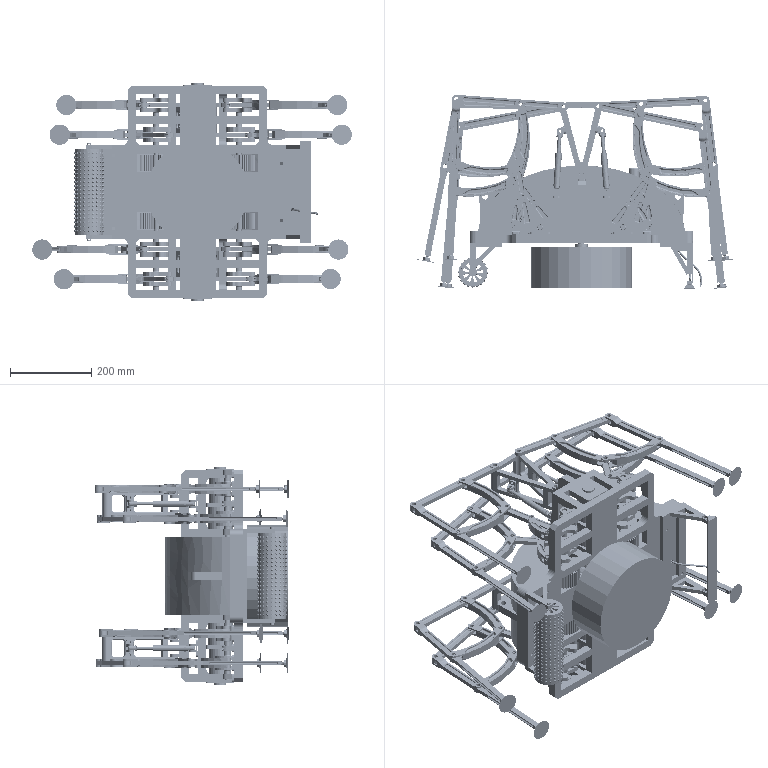Assembly | SolidWorks | mm | 149 component files | 164 solids | 12873 faces | box 787.16 x 478.96 x 537 mm | volume 15869693 mm3 | cylinder 5703 | plane 3151 | torus 1330 | cone 1064 | sphere 1040 | spline 585 | commonest cylinder face diameters 5 x964 10 x524 29.6 x390 32 x336 4 x256 6.25 x256 2 x224 3 x200
Bill of materials:
AxisSeat | 8 |  | Rounded-rectangular flange plate with two through-holes, from which a perpendicular tapered lug projects; the lug ends in a rounded boss with a large through-bore, giving a T-shaped side profile.
BallJointRod | 8 |  | Faceted sphere joined by a short cylindrical neck to a roughly square plate; the plate has a concave curved face toward the sphere and a slotted/stepped edge profile forming two parallel flanges at the back.
BallJointRodUpperPressurePlate | 8 |  | Thin rectangular plate with stepped edge profile: a wider central tongue on one face and offset tabs at the ends, producing a T-slot or tongue-like cross-section.
Rolling bearings 6302 GB 276-94 | 4 |  | Annular rolling-element unit resembling an open radial ball bearing: a plain outer ring and a plain inner ring, concentric, with a ring of spherical balls in the gap between them.
CarBody | 1 |  | Complex frame-like model: a cross-shaped plate with multiple rectangular windows, central plate with a large hole and bolt-hole pattern, stand-off rods, side brackets with triangular gussets and end eyes, a block with a cylindrical protrusion, and flexible cable-like curves.
CleaningCylinder | 1 | Flexible Polyurethane Foam | Short solid cylindrical disc with a small coaxial cylindrical pin protruding from one face.
ConnectingRod1 | 8 |  | Long slightly tapered flat bar/link with a rounded end containing a through-hole, a second through-hole midway, two shallow elongated pockets, and a semicircular cutout at the wider end flanked by small transverse holes.
ConnectingRod1-1 | 8 |  | Half-ring/saddle block: a thick curved body with a semicircular cutout, with angled or oblique holes passing through the outer curved face.
CrankshaftSeat | 8 |  | Pillow-block-like bracket: rounded-rectangular base with two through-holes at the ends and a central tapered upright with a rounded top holding a large through-bore; base underside has a shallow relief.
Cylinder | 1 |  | Cylindrical roller with a regular array of small hemispherical bumps on the outer surface, spoked open end faces (wedge-shaped windows around a hub), and a small shaft extending from both ends with small cross-holes near the shaft tips.
CylinderAxis | 4 |  | Slender cylindrical rod with an enlarged collar near one end, ending in a flat-sided tang/eye with a transverse through-hole.
CylinderBarrel | 4 |  | Cylindrical tube/body with a stepped collar near one end and a flat-sided eye end with a transverse through-hole; the opposite end appears open (hollow).
GearedMotor | 3 |  | Stacked column of two cylindrical bodies separated by square rounded-corner flanges, with a square bottom flange having corner holes, a short round boss on top, and a stepped small shaft at the bottom.
HydraulicCylinderSeat | 8 |  | Bracket: rectangular plate with rounded corners, two through-holes near its ends, and two parallel lugs sticking out from the middle. Each lug has a rounded tip and a through-hole, forming a clevis.
Leg | 8 |  | Long, slender flat bar. One end is forked into a clevis with a cross hole. There is a hole partway along the bar, a long recessed groove on the face, and a notched or grooved far end.
MainCrankshaft | 4 |  | Shaft shaped like a crankshaft: a central round shaft carrying two pairs of lobed webs. Each pair is joined by an offset cylindrical pin, and stepped journals run along the axis.
MiddleCrankshaftSeat | 4 |  | Pillow-block-style mount: base flange with rounded ends and two mounting holes, carrying a raised block with a rounded top. The block has a large through-bore parallel to the base.
RockerArm | 8 |  | Curved link arm with a forked (clevis) end at each end. Each end has paired holes, and there is a long pocket along the curved web.
ScaleInner1 | 8 |  | Curved arm with a forked end at each end and an end hole in each fork. A shaped recessed pocket runs along the curved body, and the body narrows near one end.
ScaleInner2 | 8 |  | Curved link with a forked end at each end and a hole in each tine. A shallow elongated recess runs along the top face.
ScaleInner3 | 8 |  | Straight, flat bar with rounded ends. It has a hole at each end, a central hole, and two long shallow recesses on one face.
Scraper | 1 |  | Long, slender prismatic bar whose cross-section is stepped: a narrow rectangle on top of a trapezoidal base. The top-left view shows a second offset trapezoidal outline. Small rectangular notches sit near each end.
Spring | 2 |  | Helical coil of round wire with roughly constant diameter and pitch, open coil spacing, and plain cut ends.
GB - Spur gear 2M 37T 20PA 37FW ---S37A75H50L16.0S1 | 1 |  | Spur gear: a flat cylindrical disc with straight external teeth all around and a central circular bore with a single rectangular keyway.
spur gear_gb | 4 |  | Spur gear: a flat cylindrical disc with straight external teeth and a fairly small central circular bore with a single rectangular keyway.
GB - Spur gear 2M 40T 20PA 40FW ---S40A75H50L12.0S1 | 4 |  | Spur gear: a flat cylindrical disc with straight external teeth (apparently slightly more and finer than in the other gears) and a small central circular bore with a single rectangular keyway.
SuctionCup | 8 |  | Thin circular disc with a small polygonal or rectangular boss on one face. The edge appears thin and possibly tapered.
TopCover | 1 |  | Thin-walled shroud or housing: a curved (arched) shell enclosed by end walls, with a rectangular perimeter flange around its open face. The flange has corner tabs with small holes. The lower edge has notches and a central U-shaped slot, and there is one hole in the curved wall.
UpperAxisSeat | 4 |  | Clevis-style double-lug bracket: a flat rectangular base plate with rounded corners and one through hole near each end, with two parallel, equal lugs standing up from the middle of the plate. Each lug has a rounded end, sides that taper slightly, and a large round hole; the two lug holes appear to share one axis.
VibrationDampingBracket | 2 |  | Lightweighted, truss-like triangular bracket: an open triangular frame, roughly an isosceles outline, with a round hole at each of its three rounded corners. It sits on top of a deeper structure of upright walls with large rectangular openings, diagonal braces and posts. A rectangular web in the middle carries two small holes.
Mates:
1. concentric | ScaleInner1-1 face at (-140.193, -93.224, 219.713) dir (0, 0, -1) r 5 | Leg-1 face at (-140.193, -93.224, 211.463) dir (0, 0, -1) r 5
2. coincident | ScaleInner1-1 face at (-137.996, -126.993, 201.463) dir (0, 0, 1) | Leg-1 face at (-148.968, -330.662, 201.463) dir (0, 0, -1)
3. concentric | ScaleInner1-1 face at (17.789, -104.729, 219.713) dir (0, 0, -1) r 5 | ScaleInner2-1 face at (17.789, -104.729, 215.713) dir (0, 0, -1) r 5
4. coincident | ScaleInner1-1 face at (17.789, -104.729, 197.213) dir (0, 0, 1) | ScaleInner2-1 face at (-85.717, 17.977, 197.213) dir (0, 0, -1)
5. concentric | ScaleInner3-1 face at (-134.342, 65.068, 211.463) dir (0, 0, -1) r 5 | Leg-1 face at (-134.343, 65.068, 211.463) dir (0, 0, -1) r 5
6. coincident | ScaleInner3-1 face at (128.961, 45.893, 211.463) dir (0, 0, 1) | Leg-1 face at (-134.343, 65.068, 211.463) dir (0, 0, -1)
7. concentric | ScaleInner2-1 face at (23.639, 53.563, 215.713) dir (0, 0, -1) r 5 | ScaleInner3-1 face at (23.64, 53.563, 211.463) dir (0, 0, -1) r 5
8. concentric | ConnectingRod1-1 face at (17.789, -104.729, 201.463) dir (0, 0, 1) r 5 | ScaleInner1-1 face at (17.789, -104.729, 219.713) dir (0, 0, -1) r 5
9. coincident | ConnectingRod1-1 face at (39.348, -177.229, 211.463) dir (0, 0, 1) | ScaleInner2-1 face at (51.343, -100.957, 211.463) dir (0, 0, -1)
10. concentric | ConnectingRod1-1 face at (31.955, -256.986, 206.463) dir (-0.1656, 0.9862, 0) r 1.5 | ConnectingRod1-1-1 face at (32.038, -257.479, 206.463) dir (-0.1656, 0.9862, 0) r 1.5
11. concentric | ConnectingRod1-1 face at (54.144, -253.259, 206.463) dir (-0.1656, 0.9862, 0) r 1.5 | ConnectingRod1-1-1 face at (54.227, -253.752, 206.463) dir (-0.1656, 0.9862, 0) r 1.5
12. coincident | ConnectingRod1-1 face at (72.659, -247.614, 213.963) dir (0.1656, -0.9862, 0) | ConnectingRod1-1-1 face at (28.829, -254.976, 201.463) dir (-0.1656, 0.9862, 0)
13. concentric | ConnectingRod1-1 face at (30.212, -178.693, 201.463) dir (0, 0, 1) r 5.625 | RockerArm-1 face at (30.212, -178.693, 217.463) dir (0, 0, -1) r 5.625
14. coincident | ConnectingRod1-1 face at (39.348, -177.229, 211.463) dir (0, 0, 1) | RockerArm-1 face at (67.023, -246.948, 211.463) dir (0, 0, -1)
15. concentric | CarBody-1 face at (174.617, -142.6, 213.713) dir (0, 1, 0) r 3.125 | UpperAxisSeat-1 face at (174.617, -111.1, 213.713) dir (0, -1, 0) r 3.125
16. concentric | CarBody-1 face at (174.617, -142.6, 179.213) dir (0, 1, 0) r 3.125 | UpperAxisSeat-1 face at (174.617, -111.1, 179.213) dir (0, -1, 0) r 3.125
17. coincident | CarBody-1 face at (174.617, -137.6, -8.037) dir (0, 1, 0) | UpperAxisSeat-1 face at (174.617, -137.6, 196.463) dir (0, -1, 0)
18. concentric | VibrationDampingBracket-1 face at (174.617, -120.35, 138.463) dir (0, 0, 1) r 5 | UpperAxisSeat-1 face at (174.617, -120.35, 208.463) dir (0, 0, -1) r 5
19. coincident | VibrationDampingBracket-1 face at (128.96, 45.893, 201.463) dir (0, 0, 1) | UpperAxisSeat-1 face at (174.617, -120.35, 201.463) dir (0, 0, -1)
20. concentric | CarBody-1 face at (174.617, -142.6, 126.213) dir (0, 1, 0) r 3.125 | UpperAxisSeat-2 face at (174.617, -111.1, 126.213) dir (0, -1, 0) r 3.125
21. concentric | CarBody-1 face at (174.617, -142.6, 160.713) dir (0, 1, 0) r 3.125 | UpperAxisSeat-2 face at (174.617, -111.1, 160.713) dir (0, -1, 0) r 3.125
22. coincident | CarBody-1 face at (174.617, -137.6, -8.037) dir (0, 1, 0) | UpperAxisSeat-2 face at (174.617, -137.6, 143.463) dir (0, -1, 0)
23. concentric | CarBody-1 face at (12.617, -274.1, 220.838) dir (0, 1, 0) r 3.125 | AxisSeat-1 face at (12.617, -266.35, 220.838) dir (0, 1, 0) r 4.5
24. concentric | CarBody-1 face at (12.617, -274.1, 192.088) dir (0, 1, 0) r 3.125 | AxisSeat-1 face at (12.617, -266.35, 192.088) dir (0, 1, 0) r 4.5
25. coincident | CarBody-1 face at (449.617, -269.1, -108.037) dir (0, 1, 0) | AxisSeat-1 face at (12.617, -269.1, 206.463) dir (0, -1, 0)
26. concentric | RockerArm-1 face at (12.617, -251.6, 217.463) dir (0, 0, -1) r 5.625 | AxisSeat-1 face at (12.617, -251.6, 201.463) dir (0, 0, 1) r 5.625
27. coincident | RockerArm-1 face at (56.993, -257.493, 211.463) dir (0, 0, -1) | AxisSeat-1 face at (12.617, -251.6, 211.463) dir (0, 0, 1)
28. concentric | ScaleInner3-1 face at (128.961, 45.893, 211.463) dir (0, 0, -1) r 5 | VibrationDampingBracket-1 face at (128.96, 45.893, 138.463) dir (0, 0, 1) r 5
29. concentric | CarBody-1 face at (52.617, -274.1, 242.963) dir (0, 1, 0) r 3.125 | CrankshaftSeat-1 face at (52.617, -269.1, 242.963) dir (0, 1, 0) r 3.125
30. concentric | CarBody-1 face at (92.617, -274.1, 242.963) dir (0, 1, 0) r 3.125 | CrankshaftSeat-1 face at (92.617, -269.1, 242.963) dir (0, 1, 0) r 3.125
31. coincident | CarBody-1 face at (449.617, -269.1, -108.037) dir (0, 1, 0) | CrankshaftSeat-1 face at (72.617, -269.1, 242.963) dir (0, -1, 0)
32. concentric | CarBody-1 face at (52.617, -274.1, 96.963) dir (0, 1, 0) r 3.125 | CrankshaftSeat-2 face at (52.617, -269.1, 96.963) dir (0, 1, 0) r 3.125
33. concentric | CarBody-1 face at (92.617, -274.1, 96.963) dir (0, 1, 0) r 3.125 | CrankshaftSeat-2 face at (92.617, -269.1, 96.963) dir (0, 1, 0) r 3.125
34. coincident | CarBody-1 face at (449.617, -269.1, -108.037) dir (0, 1, 0) | CrankshaftSeat-2 face at (72.617, -269.1, 96.963) dir (0, -1, 0)
35. concentric | MainCrankshaft-1 face at (72.617, -251.6, 247.963) dir (0, 0, -1) r 6.75 | CrankshaftSeat-1 face at (72.617, -251.6, 239.963) dir (0, 0, 1) r 6.75
36. concentric | ConnectingRod1-1 face at (42.635, -252.657, 201.463) dir (0, 0, 1) r 7.5 | MainCrankshaft-1 face at (42.635, -252.657, 213.963) dir (0, 0, -1) r 6.25
37. concentric | Leg-2 face at (-144.409, -161.167, 138.463) dir (0, 0, -1) r 5 | ScaleInner1-2 face at (-144.409, -161.167, 146.713) dir (0, 0, -1) r 5
38. concentric | ScaleInner3-2 face at (-130.399, -3.388, 138.463) dir (0, 0, -1) r 5 | Leg-2 face at (-130.399, -3.388, 138.463) dir (0, 0, -1) r 5
39. coincident | ScaleInner3-2 face at (128.961, 45.893, 138.463) dir (0, 0, 1) | Leg-2 face at (-130.399, -3.388, 138.463) dir (0, 0, -1)
40. concentric | ScaleInner3-2 face at (25.217, 26.181, 138.463) dir (0, 0, -1) r 5 | ScaleInner2-2 face at (25.216, 26.181, 142.713) dir (0, 0, -1) r 5
41. coincident | ScaleInner3-2 face at (128.961, 45.893, 138.463) dir (0, 0, 1) | ScaleInner2-2 face at (25.216, 26.181, 138.463) dir (0, 0, -1)
42. coincident | Leg-2 face at (-165.423, -397.836, 128.463) dir (0, 0, -1) | ScaleInner1-2 face at (-133.59, -193.232, 128.463) dir (0, 0, 1)
43. concentric | ScaleInner1-2 face at (11.207, -131.599, 146.713) dir (0, 0, -1) r 5 | ScaleInner2-2 face at (11.207, -131.599, 142.713) dir (0, 0, -1) r 5
44. concentric | ConnectingRod1-2 face at (95.201, -259.379, 133.463) dir (-0.6093, 0.793, 0) r 1.5 | ConnectingRod1-1-2 face at (95.505, -259.776, 133.463) dir (-0.6093, 0.793, 0) r 1.5
45. concentric | ConnectingRod1-2 face at (113.042, -245.671, 133.463) dir (-0.6093, 0.793, 0) r 1.5 | ConnectingRod1-1-2 face at (113.347, -246.067, 133.463) dir (-0.6093, 0.793, 0) r 1.5
46. coincident | ConnectingRod1-2 face at (126.739, -231.994, 140.963) dir (0.6093, -0.793, 0) | ConnectingRod1-1-2 face at (91.497, -259.072, 128.463) dir (-0.6093, 0.793, 0)
47. concentric | ConnectingRod1-2 face at (56.903, -191.071, 128.463) dir (0, 0, 1) r 5.625 | RockerArm-2 face at (56.903, -191.071, 144.463) dir (0, 0, -1) r 5.625
48. coincident | ConnectingRod1-2 face at (64.282, -185.489, 138.463) dir (0, 0, 1) | RockerArm-2 face at (64.626, -268.234, 138.463) dir (0, 0, -1)
49. concentric | ConnectingRod1-2 face at (11.207, -131.599, 128.463) dir (0, 0, 1) r 5 | ScaleInner2-2 face at (11.207, -131.599, 142.713) dir (0, 0, -1) r 5
50. coincident | ConnectingRod1-2 face at (64.282, -185.489, 138.463) dir (0, 0, 1) | ScaleInner2-2 face at (44.911, -129.563, 138.463) dir (0, 0, -1)
51. concentric | VibrationDampingBracket-1 face at (128.96, 45.893, 138.463) dir (0, 0, 1) r 5 | ScaleInner3-2 face at (128.961, 45.893, 138.463) dir (0, 0, -1) r 5
52. coincident | VibrationDampingBracket-1 face at (128.96, 45.893, 138.463) dir (0, 0, -1) | ScaleInner3-2 face at (128.961, 45.893, 138.463) dir (0, 0, 1)
53. concentric | MainCrankshaft-1 face at (102.598, -250.543, 140.963) dir (0, 0, -1) r 6.25 | ConnectingRod1-2 face at (102.598, -250.543, 128.463) dir (0, 0, 1) r 7.5
54. concentric | CarBody-1 face at (12.617, -274.1, 147.838) dir (0, 1, 0) r 3.125 | AxisSeat-2 face at (12.617, -266.35, 147.838) dir (0, 1, 0) r 4.5
55. concentric | CarBody-1 face at (12.617, -274.1, 119.088) dir (0, 1, 0) r 3.125 | AxisSeat-2 face at (12.617, -242.85, 119.088) dir (0, -1, 0) r 3.125
56. coincident | CarBody-1 face at (449.617, -269.1, -108.037) dir (0, 1, 0) | AxisSeat-2 face at (12.617, -269.1, 133.463) dir (0, -1, 0)
57. concentric | RockerArm-2 face at (12.617, -251.6, 144.463) dir (0, 0, -1) r 5.625 | AxisSeat-2 face at (12.617, -251.6, 138.463) dir (0, 0, -1) r 5.625
58. concentric | CarBody-1 face at (48.617, -274.1, 169.963) dir (0, 1, 0) r 3.125 | MiddleCrankshaftSeat-1 face at (48.617, -262.85, 169.963) dir (0, -1, 0) r 3.125
59. concentric | CarBody-1 face at (96.617, -274.1, 169.963) dir (0, 1, 0) r 3.125 | MiddleCrankshaftSeat-1 face at (96.617, -262.85, 169.963) dir (0, -1, 0) r 3.125
60. coincident | CarBody-1 face at (449.617, -269.1, -108.037) dir (0, 1, 0) | MiddleCrankshaftSeat-1 face at (72.617, -269.1, 169.963) dir (0, -1, 0)
61. coincident | MainCrankshaft-1 face at (72.617, -251.6, 106.963) dir (0, 0, -1) | CrankshaftSeat-2 face at (47.617, -262.85, 106.963) dir (0, 0, 1)
62. concentric | ConnectingRod1-3 face at (54.284, -247.009, -149.537) dir (-0.3125, 0.9499, 0) r 1.5 | ConnectingRod1-1-5 face at (54.44, -247.484, -149.537) dir (-0.3125, 0.9499, 0) r 1.5
63. concentric | ConnectingRod1-3 face at (32.91, -254.04, -149.537) dir (-0.3125, 0.9499, 0) r 1.5 | ConnectingRod1-1-5 face at (33.067, -254.515, -149.537) dir (-0.3125, 0.9499, 0) r 1.5
64. coincident | ConnectingRod1-3 face at (71.736, -238.637, -142.037) dir (0.3125, -0.9499, 0) | ConnectingRod1-1-5 face at (49.94, -245.806, -154.537) dir (-0.3125, 0.9499, 0)
65. concentric | ConnectingRod1-1-4 face at (235.786, -248.339, 206.463) dir (0.5913, 0.8065, 0) r 1.5 | ConnectingRod1-4 face at (236.082, -247.936, 206.463) dir (0.5913, 0.8065, 0) r 1.5
66. concentric | ConnectingRod1-1-4 face at (253.932, -261.642, 206.463) dir (0.5913, 0.8065, 0) r 1.5 | ConnectingRod1-4 face at (254.227, -261.239, 206.463) dir (0.5913, 0.8065, 0) r 1.5
67. coincident | ConnectingRod1-1-4 face at (240.584, -248.137, 211.463) dir (0.5913, 0.8065, 0) | ConnectingRod1-4 face at (222.08, -234.571, 198.963) dir (-0.5913, -0.8065, 0)
68. concentric | Leg-3 face at (-162.383, -100.897, -144.537) dir (0, 0, -1) r 5 | ScaleInner1-3 face at (-162.383, -100.897, -136.287) dir (0, 0, -1) r 5
69. coincident | Leg-3 face at (-207.807, -334.115, -144.537) dir (0, 0, 1) | ScaleInner1-3 face at (-158.75, -134.542, -144.537) dir (0, 0, -1)
70. concentric | ScaleInner2-3 face at (-4.055, -105.661, -140.287) dir (0, 0, -1) r 5 | ScaleInner1-3 face at (-4.055, -105.661, -136.287) dir (0, 0, -1) r 5
71. coincident | ScaleInner2-3 face at (-87.318, 31.589, -140.287) dir (0, 0, 1) | ScaleInner1-3 face at (-4.055, -105.661, -140.287) dir (0, 0, -1)
72. concentric | ScaleInner3-3 face at (-132.1, 54.581, -144.537) dir (0, 0, -1) r 5 | Leg-3 face at (-132.1, 54.581, -144.537) dir (0, 0, -1) r 5
73. coincident | ScaleInner3-3 face at (131.781, 46.642, -144.537) dir (0, 0, 1) | Leg-3 face at (-132.1, 54.581, -144.537) dir (0, 0, -1)
74. concentric | ScaleInner3-3 face at (26.228, 49.818, -144.537) dir (0, 0, -1) r 5 | ScaleInner2-3 face at (26.228, 49.818, -140.287) dir (0, 0, -1) r 5
75. concentric | ScaleInner2-3 face at (-4.055, -105.661, -140.287) dir (0, 0, -1) r 5 | ConnectingRod1-3 face at (-4.055, -105.661, -154.537) dir (0, 0, 1) r 5
76. coincident | ScaleInner2-3 face at (29.679, -107.129, -144.537) dir (0, 0, -1) | ConnectingRod1-3 face at (28.191, -174.08, -144.537) dir (0, 0, 1)
77. concentric | CarBody-1 face at (174.617, -142.6, -142.287) dir (0, 1, 0) r 3.125 | UpperAxisSeat-3 face at (174.617, -111.1, -142.287) dir (0, -1, 0) r 3.125
78. concentric | CarBody-1 face at (174.617, -142.6, -176.787) dir (0, 1, 0) r 3.125 | UpperAxisSeat-3 face at (174.617, -111.1, -176.787) dir (0, -1, 0) r 3.125
79. coincident | CarBody-1 face at (174.617, -137.6, -8.037) dir (0, 1, 0) | UpperAxisSeat-3 face at (174.617, -137.6, -159.537) dir (0, -1, 0)
80. concentric | CarBody-1 face at (174.617, -142.6, -195.287) dir (0, 1, 0) r 3.125 | UpperAxisSeat-4 face at (174.617, -111.1, -195.287) dir (0, -1, 0) r 3.125
81. concentric | CarBody-1 face at (174.617, -142.6, -229.787) dir (0, 1, 0) r 3.125 | UpperAxisSeat-4 face at (174.617, -111.1, -229.787) dir (0, -1, 0) r 3.125
82. coincident | CarBody-1 face at (174.617, -137.6, -8.037) dir (0, 1, 0) | UpperAxisSeat-4 face at (174.617, -137.6, -212.537) dir (0, -1, 0)
83. concentric | UpperAxisSeat-4 face at (174.617, -120.35, -224.537) dir (0, 0, 1) r 5 | VibrationDampingBracket-2 face at (174.617, -120.35, -217.537) dir (0, 0, 1) r 5
84. coincident | UpperAxisSeat-4 face at (174.617, -120.35, -217.537) dir (0, 0, 1) | VibrationDampingBracket-2 face at (131.78, 46.642, -217.537) dir (0, 0, -1)
85. concentric | ScaleInner3-3 face at (131.781, 46.642, -144.537) dir (0, 0, -1) r 5 | VibrationDampingBracket-2 face at (131.78, 46.642, -217.537) dir (0, 0, 1) r 5
86. coincident | ScaleInner3-3 face at (131.781, 46.642, -154.537) dir (0, 0, -1) | VibrationDampingBracket-2 face at (131.78, 46.642, -154.537) dir (0, 0, 1)
87. coincident | Leg-4 face at (-127.342, -3.874, -217.537) dir (0, 0, -1) | ScaleInner3-4 face at (131.781, 46.642, -217.537) dir (0, 0, 1)
88. concentric | Leg-4 face at (-127.342, -3.874, -217.537) dir (0, 0, -1) r 5 | ScaleInner3-4 face at (-127.341, -3.874, -217.537) dir (0, 0, -1) r 5
89. concentric | VibrationDampingBracket-2 face at (131.78, 46.642, -217.537) dir (0, 0, 1) r 5 | ScaleInner3-4 face at (131.781, 46.642, -217.537) dir (0, 0, -1) r 5
90. coincident | VibrationDampingBracket-2 face at (131.78, 46.642, -217.537) dir (0, 0, -1) | ScaleInner3-4 face at (131.781, 46.642, -217.537) dir (0, 0, 1)
91. concentric | ConnectingRod1-3 face at (19.381, -176.905, -154.537) dir (0, 0, 1) r 5.625 | RockerArm-4 face at (19.381, -176.905, -138.037) dir (0, 0, -1) r 5.625
92. coincident | ConnectingRod1-3 face at (28.191, -174.08, -154.537) dir (0, 0, -1) | RockerArm-4 face at (65.761, -239.055, -154.537) dir (0, 0, 1)
93. concentric | CarBody-1 face at (52.617, -274.1, -113.037) dir (0, 1, 0) r 3.125 | CrankshaftSeat-3 face at (52.617, -269.1, -113.037) dir (0, 1, 0) r 3.125
94. concentric | CarBody-1 face at (92.617, -274.1, -113.037) dir (0, 1, 0) r 3.125 | CrankshaftSeat-3 face at (92.617, -269.1, -113.037) dir (0, 1, 0) r 3.125
95. coincident | CarBody-1 face at (449.617, -269.1, -108.037) dir (0, 1, 0) | CrankshaftSeat-3 face at (72.617, -269.1, -113.037) dir (0, -1, 0)
96. concentric | CarBody-1 face at (52.617, -274.1, -259.037) dir (0, 1, 0) r 3.125 | CrankshaftSeat-4 face at (52.617, -269.1, -259.037) dir (0, 1, 0) r 3.125
97. concentric | CarBody-1 face at (92.617, -274.1, -259.037) dir (0, 1, 0) r 3.125 | CrankshaftSeat-4 face at (92.617, -269.1, -259.037) dir (0, 1, 0) r 3.125
98. coincident | CarBody-1 face at (449.617, -269.1, -108.037) dir (0, 1, 0) | CrankshaftSeat-4 face at (72.617, -269.1, -259.037) dir (0, -1, 0)
99. concentric | CarBody-1 face at (12.617, -274.1, -135.162) dir (0, 1, 0) r 3.125 | AxisSeat-3 face at (12.617, -266.35, -135.162) dir (0, 1, 0) r 4.5
100. concentric | CarBody-1 face at (12.617, -274.1, -163.912) dir (0, 1, 0) r 3.125 | AxisSeat-3 face at (12.617, -242.85, -163.912) dir (0, -1, 0) r 3.125
101. coincident | CarBody-1 face at (449.617, -269.1, -108.037) dir (0, 1, 0) | AxisSeat-3 face at (12.617, -269.1, -149.537) dir (0, -1, 0)
102. concentric | CarBody-1 face at (12.617, -274.1, -236.912) dir (0, 1, 0) r 3.125 | AxisSeat-4 face at (12.617, -242.85, -236.912) dir (0, -1, 0) r 3.125
103. concentric | CarBody-1 face at (12.617, -274.1, -208.162) dir (0, 1, 0) r 3.125 | AxisSeat-4 face at (12.617, -242.85, -208.162) dir (0, -1, 0) r 3.125
104. coincident | CarBody-1 face at (449.617, -269.1, -108.037) dir (0, 1, 0) | AxisSeat-4 face at (12.617, -269.1, -222.537) dir (0, -1, 0)
105. concentric | RockerArm-4 face at (12.617, -251.6, -138.037) dir (0, 0, -1) r 5.625 | AxisSeat-3 face at (12.617, -251.6, -144.537) dir (0, 0, -1) r 5.625
106. concentric | CrankshaftSeat-4 face at (72.617, -251.6, -262.037) dir (0, 0, 1) r 6.75 | MainCrankshaft-3 face at (72.617, -251.6, -264.037) dir (0, 0, 1) r 6.75
107. concentric | ConnectingRod1-1-5 face at (42.816, -248.15, -154.537) dir (0, 0, 1) r 7.5 | MainCrankshaft-3 face at (42.816, -248.15, -157.037) dir (0, 0, 1) r 6.25
108. concentric | CarBody-1 face at (48.617, -274.1, -186.037) dir (0, 1, 0) r 3.125 | MiddleCrankshaftSeat-2 face at (48.617, -262.85, -186.037) dir (0, -1, 0) r 3.125
109. concentric | CarBody-1 face at (96.617, -274.1, -186.037) dir (0, 1, 0) r 3.125 | MiddleCrankshaftSeat-2 face at (96.617, -262.85, -186.037) dir (0, -1, 0) r 3.125
110. coincident | CarBody-1 face at (449.617, -269.1, -108.037) dir (0, 1, 0) | MiddleCrankshaftSeat-2 face at (72.617, -269.1, -186.037) dir (0, -1, 0)
111. width | MainCrankshaft-3 face at (72.617, -251.6, -178.537) dir (0, 0, -1) | MainCrankshaft-3 face at (72.617, -251.6, -193.537) dir (0, 0, 1) | MiddleCrankshaftSeat-2 face at (72.617, -251.6, -192.287) dir (0, 0, -1) | MiddleCrankshaftSeat-2 face at (72.617, -251.6, -179.787) dir (0, 0, 1)
112. concentric | ScaleInner1-5 face at (490.257, -164.548, 193.213) dir (0, 0, 1) r 5 | Leg-5 face at (490.257, -164.548, 201.463) dir (0, 0, 1) r 5
113. coincident | ScaleInner1-5 face at (478.742, -196.369, 201.463) dir (0, 0, 1) | Leg-5 face at (518.366, -400.479, 201.463) dir (0, 0, -1)
114. concentric | ScaleInner2-5 face at (335.321, -131.599, 215.713) dir (0, 0, -1) r 5 | ScaleInner1-5 face at (335.321, -131.599, 193.213) dir (0, 0, 1) r 5
115. coincident | ScaleInner2-5 face at (437.845, -79.504, 197.213) dir (0, 0, -1) | ScaleInner1-5 face at (335.321, -131.599, 197.213) dir (0, 0, 1)
116. concentric | ScaleInner3-5 face at (471.517, -7.26, 201.463) dir (0, 0, 1) r 5 | Leg-5 face at (471.517, -7.26, 201.463) dir (0, 0, 1) r 5
117. coincident | ScaleInner3-5 face at (213.291, 47.655, 201.463) dir (0, 0, -1) | Leg-5 face at (471.517, -7.26, 201.463) dir (0, 0, 1)
118. concentric | ScaleInner2-5 face at (316.582, 25.689, 215.713) dir (0, 0, -1) r 5 | ScaleInner3-5 face at (316.582, 25.689, 201.463) dir (0, 0, 1) r 5
119. concentric | ConnectingRod1-4 face at (335.321, -131.599, 211.463) dir (0, 0, -1) r 5 | ScaleInner2-5 face at (335.321, -131.599, 215.713) dir (0, 0, -1) r 5
120. coincident | ConnectingRod1-4 face at (283.474, -186.671, 211.463) dir (0, 0, 1) | ScaleInner2-5 face at (335.321, -131.599, 211.463) dir (0, 0, -1)
121. concentric | Leg-6 face at (499.558, -96.509, 128.463) dir (0, 0, 1) r 5 | ScaleInner1-6 face at (499.558, -96.509, 120.213) dir (0, 0, 1) r 5
122. coincident | Leg-6 face at (529.232, -332.248, 128.463) dir (0, 0, -1) | ScaleInner1-6 face at (496.657, -130.224, 128.463) dir (0, 0, 1)
123. concentric | ScaleInner2-6 face at (341.371, -104.714, 142.713) dir (0, 0, -1) r 5 | ScaleInner1-6 face at (341.371, -104.714, 120.213) dir (0, 0, 1) r 5
124. coincident | ScaleInner2-6 face at (443.546, -51.94, 124.213) dir (0, 0, -1) | ScaleInner1-6 face at (341.371, -104.714, 124.213) dir (0, 0, 1)
125. concentric | ScaleInner3-6 face at (479.775, 60.651, 128.463) dir (0, 0, 1) r 5 | Leg-6 face at (479.775, 60.651, 128.463) dir (0, 0, 1) r 5
126. coincident | ScaleInner3-6 face at (216.129, 46.976, 128.463) dir (0, 0, -1) | Leg-6 face at (479.775, 60.651, 128.463) dir (0, 0, 1)
127. concentric | ScaleInner3-6 face at (321.587, 52.446, 128.463) dir (0, 0, 1) r 5 | ScaleInner2-6 face at (321.588, 52.446, 142.713) dir (0, 0, -1) r 5
128. concentric | VibrationDampingBracket-2 face at (216.129, 46.976, -217.537) dir (0, 0, 1) r 5 | ScaleInner3-6 face at (216.129, 46.976, 128.463) dir (0, 0, 1) r 5
129. coincident | VibrationDampingBracket-1 face at (128.96, 45.893, 138.463) dir (0, 0, -1) | ScaleInner3-6 face at (216.129, 46.976, 138.463) dir (0, 0, 1)
130. concentric | VibrationDampingBracket-1 face at (213.292, 47.655, 138.463) dir (0, 0, 1) r 5 | ScaleInner3-5 face at (213.291, 47.655, 201.463) dir (0, 0, 1) r 5
131. coincident | VibrationDampingBracket-1 face at (128.96, 45.893, 201.463) dir (0, 0, 1) | ScaleInner3-5 face at (213.291, 47.655, 201.463) dir (0, 0, -1)
132. concentric | ConnectingRod1-4 face at (290.977, -192.085, 211.463) dir (0, 0, -1) r 5.625 | RockerArm-6 face at (290.977, -192.085, 194.963) dir (0, 0, 1) r 5.625
133. concentric | CarBody-1 face at (296.617, -274.1, 242.963) dir (0, 1, 0) r 3.125 | CrankshaftSeat-5 face at (296.617, -269.1, 242.963) dir (0, 1, 0) r 3.125
134. concentric | CarBody-1 face at (256.617, -274.1, 242.963) dir (0, 1, 0) r 3.125 | CrankshaftSeat-5 face at (256.617, -269.1, 242.963) dir (0, 1, 0) r 3.125
135. coincident | CarBody-1 face at (449.617, -269.1, -108.037) dir (0, 1, 0) | CrankshaftSeat-5 face at (276.617, -269.1, 242.963) dir (0, -1, 0)
136. concentric | CarBody-1 face at (296.617, -274.1, 96.963) dir (0, 1, 0) r 3.125 | CrankshaftSeat-6 face at (296.617, -269.1, 96.963) dir (0, 1, 0) r 3.125
137. concentric | CarBody-1 face at (256.617, -274.1, 96.963) dir (0, 1, 0) r 3.125 | CrankshaftSeat-6 face at (256.617, -269.1, 96.963) dir (0, 1, 0) r 3.125
138. coincident | CarBody-1 face at (449.617, -269.1, -108.037) dir (0, 1, 0) | CrankshaftSeat-6 face at (276.617, -269.1, 96.963) dir (0, -1, 0)
139. concentric | CarBody-1 face at (336.617, -274.1, 220.838) dir (0, 1, 0) r 3.125 | AxisSeat-5 face at (336.617, -266.35, 220.838) dir (0, 1, 0) r 4.5
140. concentric | CarBody-1 face at (336.617, -274.1, 192.088) dir (0, 1, 0) r 3.125 | AxisSeat-5 face at (336.617, -266.35, 192.088) dir (0, 1, 0) r 4.5
141. coincident | CarBody-1 face at (449.617, -269.1, -108.037) dir (0, 1, 0) | AxisSeat-5 face at (336.617, -269.1, 206.463) dir (0, -1, 0)
142. concentric | CarBody-1 face at (336.617, -274.1, 119.088) dir (0, 1, 0) r 3.125 | AxisSeat-6 face at (336.617, -266.35, 119.088) dir (0, 1, 0) r 4.5
143. concentric | CarBody-1 face at (336.617, -274.1, 147.838) dir (0, 1, 0) r 3.125 | AxisSeat-6 face at (336.617, -266.35, 147.838) dir (0, 1, 0) r 4.5
144. coincident | CarBody-1 face at (449.617, -269.1, -108.037) dir (0, 1, 0) | AxisSeat-6 face at (336.617, -269.1, 133.463) dir (0, -1, 0)
145. concentric | CarBody-1 face at (300.617, -274.1, 169.963) dir (0, 1, 0) r 3.125 | MiddleCrankshaftSeat-3 face at (300.617, -262.85, 169.963) dir (0, -1, 0) r 3.125
146. concentric | CarBody-1 face at (252.617, -274.1, 169.963) dir (0, 1, 0) r 3.125 | MiddleCrankshaftSeat-3 face at (252.617, -262.85, 169.963) dir (0, -1, 0) r 3.125
147. coincident | CarBody-1 face at (449.617, -269.1, -108.037) dir (0, 1, 0) | MiddleCrankshaftSeat-3 face at (276.617, -269.1, 169.963) dir (0, -1, 0)
148. concentric | CrankshaftSeat-5 face at (276.617, -251.6, 239.963) dir (0, 0, 1) r 6.75 | MainCrankshaft-4 face at (276.617, -251.6, 247.963) dir (0, 0, -1) r 6.75
149. coincident | ConnectingRod1-4 face at (283.474, -186.671, 211.463) dir (0, 0, 1) | RockerArm-6 face at (284.996, -269.403, 211.463) dir (0, 0, -1)
150. concentric | RockerArm-6 face at (336.617, -251.6, 194.963) dir (0, 0, 1) r 5.625 | AxisSeat-5 face at (336.617, -251.6, 201.463) dir (0, 0, 1) r 5.625
151. concentric | RockerArm-5 face at (336.617, -251.6, 121.963) dir (0, 0, 1) r 5.625 | AxisSeat-6 face at (336.617, -251.6, 128.463) dir (0, 0, 1) r 5.625
152. concentric | ConnectingRod1-1-4 face at (246.633, -252.571, 211.463) dir (0, 0, -1) r 7.5 | MainCrankshaft-4 face at (246.633, -252.571, 213.963) dir (0, 0, -1) r 6.25
153. concentric | ConnectingRod1-1-6 face at (294.962, -250.939, 133.463) dir (0.2318, 0.9728, 0) r 1.5 | ConnectingRod1-7 face at (295.078, -250.453, 133.463) dir (0.2318, 0.9728, 0) r 1.5
154. concentric | ConnectingRod1-1-6 face at (316.849, -256.154, 133.463) dir (0.2318, 0.9728, 0) r 1.5 | ConnectingRod1-7 face at (316.965, -255.668, 133.463) dir (0.2318, 0.9728, 0) r 1.5
155. coincident | ConnectingRod1-1-6 face at (313.897, -252.367, 128.463) dir (0.2318, 0.9728, 0) | ConnectingRod1-7 face at (276.986, -243.571, 125.963) dir (-0.2318, -0.9728, 0)
156. concentric | RockerArm-5 face at (323.986, -177.671, 121.963) dir (0, 0, 1) r 5.625 | ConnectingRod1-7 face at (323.986, -177.671, 138.463) dir (0, 0, -1) r 5.625
157. concentric | ScaleInner2-6 face at (341.371, -104.714, 142.713) dir (0, 0, -1) r 5 | ConnectingRod1-7 face at (341.371, -104.714, 138.463) dir (0, 0, -1) r 5
158. coincident | RockerArm-5 face at (282.649, -243.284, 138.463) dir (0, 0, -1) | ConnectingRod1-7 face at (314.97, -175.594, 138.463) dir (0, 0, 1)
159. coincident | RockerArm-5 face at (291.944, -254.482, 127.963) dir (0, 0, 1) | AxisSeat-6 face at (336.617, -251.6, 128.463) dir (0, 0, -1)
160. concentric | ConnectingRod1-1-6 face at (306.601, -250.628, 128.463) dir (0, 0, 1) r 7.5 | MainCrankshaft-4 face at (306.601, -250.628, 140.963) dir (0, 0, -1) r 6.25
161. width | MiddleCrankshaftSeat-3 face at (276.617, -251.6, 176.213) dir (0, 0, 1) | MiddleCrankshaftSeat-3 face at (276.617, -251.6, 163.713) dir (0, 0, -1) | MainCrankshaft-4 face at (276.617, -251.6, 177.463) dir (0, 0, -1) | MainCrankshaft-4 face at (276.617, -251.6, 162.463) dir (0, 0, 1)
162. concentric | ScaleInner3-7 face at (479.643, 62.982, -227.537) dir (0, 0, 1) r 5 | Leg-7 face at (479.644, 62.982, -217.537) dir (0, 0, -1) r 5
163. concentric | ConnectingRod1-8 face at (295.086, -253.542, -222.537) dir (0.159, 0.9873, 0) r 1.5 | ConnectingRod1-1-8 face at (295.006, -254.036, -222.537) dir (0.159, 0.9873, 0) r 1.5
164. concentric | ConnectingRod1-8 face at (317.3, -257.12, -222.537) dir (0.159, 0.9873, 0) r 1.5 | ConnectingRod1-1-8 face at (317.22, -257.613, -222.537) dir (0.159, 0.9873, 0) r 1.5
165. coincident | ConnectingRod1-8 face at (276.533, -248.022, -230.037) dir (-0.159, -0.9873, 0) | ConnectingRod1-1-8 face at (320.412, -255.089, -217.537) dir (0.159, 0.9873, 0)
166. concentric | ConnectingRod1-8 face at (318.516, -178.817, -217.537) dir (0, 0, -1) r 5.625 | RockerArm-7 face at (318.516, -178.817, -234.037) dir (0, 0, 1) r 5.625
167. coincident | ConnectingRod1-8 face at (309.37, -177.414, -217.537) dir (0, 0, 1) | RockerArm-7 face at (282.18, -247.326, -217.537) dir (0, 0, -1)
168. concentric | ScaleInner3-8 face at (474.71, -6.24, -144.537) dir (0, 0, -1) r 5 | Leg-8 face at (474.71, -6.241, -144.537) dir (0, 0, -1) r 5
169. coincident | ScaleInner3-8 face at (216.129, 46.976, -144.537) dir (0, 0, 1) | Leg-8 face at (474.71, -6.241, -144.537) dir (0, 0, -1)
170. concentric | Leg-8 face at (493.45, -163.528, -144.537) dir (0, 0, -1) r 5 | ScaleInner1-8 face at (493.45, -163.528, -162.787) dir (0, 0, 1) r 5
171. coincident | Leg-8 face at (521.559, -399.46, -154.537) dir (0, 0, -1) | ScaleInner1-8 face at (482.145, -195.425, -154.537) dir (0, 0, 1)
172. concentric | ScaleInner3-8 face at (319.561, 25.689, -144.537) dir (0, 0, -1) r 5 | ScaleInner2-8 face at (319.562, 25.689, -140.287) dir (0, 0, -1) r 5
173. coincident | ScaleInner3-8 face at (216.129, 46.976, -144.537) dir (0, 0, 1) | ScaleInner2-8 face at (286.997, 16.766, -144.537) dir (0, 0, -1)
174. concentric | ScaleInner2-8 face at (338.301, -131.598, -140.287) dir (0, 0, -1) r 5 | ScaleInner1-8 face at (338.301, -131.598, -162.787) dir (0, 0, 1) r 5
175. concentric | ScaleInner2-8 face at (338.301, -131.598, -140.287) dir (0, 0, -1) r 5 | ConnectingRod1-9 face at (338.301, -131.598, -154.537) dir (0, 0, 1) r 5
176. coincident | ScaleInner2-8 face at (338.301, -131.598, -154.537) dir (0, 0, 1) | ConnectingRod1-9 face at (299.754, -196.676, -154.537) dir (0, 0, -1)
177. concentric | ConnectingRod1-9 face at (236.21, -245.442, -149.537) dir (0.6111, 0.7916, 0) r 1.5 | ConnectingRod1-1-9 face at (235.905, -245.837, -149.537) dir (0.6111, 0.7916, 0) r 1.5
178. concentric | ConnectingRod1-9 face at (254.021, -259.19, -149.537) dir (0.6111, 0.7916, 0) r 1.5 | ConnectingRod1-1-9 face at (253.716, -259.586, -149.537) dir (0.6111, 0.7916, 0) r 1.5
179. coincident | ConnectingRod1-9 face at (270.743, -268.94, -142.037) dir (-0.6111, -0.7916, 0) | ConnectingRod1-1-9 face at (252.58, -254.92, -154.537) dir (0.6111, 0.7916, 0)
180. concentric | CarBody-1 face at (296.617, -274.1, -259.037) dir (0, 1, 0) r 3.125 | CrankshaftSeat-7 face at (296.617, -269.1, -259.037) dir (0, 1, 0) r 3.125
181. concentric | CarBody-1 face at (256.617, -274.1, -259.037) dir (0, 1, 0) r 3.125 | CrankshaftSeat-7 face at (256.617, -269.1, -259.037) dir (0, 1, 0) r 3.125
182. coincident | CarBody-1 face at (449.617, -269.1, -108.037) dir (0, 1, 0) | CrankshaftSeat-7 face at (276.617, -269.1, -259.037) dir (0, -1, 0)
183. concentric | CarBody-1 face at (256.617, -274.1, -113.037) dir (0, 1, 0) r 3.125 | CrankshaftSeat-8 face at (256.617, -269.1, -113.037) dir (0, 1, 0) r 3.125
184. concentric | CarBody-1 face at (296.617, -274.1, -113.037) dir (0, 1, 0) r 3.125 | CrankshaftSeat-8 face at (296.617, -269.1, -113.037) dir (0, 1, 0) r 3.125
185. coincident | CarBody-1 face at (449.617, -269.1, -108.037) dir (0, 1, 0) | CrankshaftSeat-8 face at (276.617, -269.1, -113.037) dir (0, -1, 0)
186. concentric | CarBody-1 face at (336.617, -274.1, -236.912) dir (0, 1, 0) r 3.125 | AxisSeat-7 face at (336.617, -266.35, -236.912) dir (0, 1, 0) r 4.5
187. concentric | CarBody-1 face at (336.617, -274.1, -208.162) dir (0, 1, 0) r 3.125 | AxisSeat-7 face at (336.617, -266.35, -208.162) dir (0, 1, 0) r 4.5
188. coincident | CarBody-1 face at (449.617, -269.1, -108.037) dir (0, 1, 0) | AxisSeat-7 face at (336.617, -269.1, -222.537) dir (0, -1, 0)
189. concentric | CarBody-1 face at (336.617, -274.1, -135.162) dir (0, 1, 0) r 3.125 | AxisSeat-8 face at (336.617, -266.35, -135.162) dir (0, 1, 0) r 4.5
190. concentric | CarBody-1 face at (336.617, -274.1, -163.912) dir (0, 1, 0) r 3.125 | AxisSeat-8 face at (336.617, -266.35, -163.912) dir (0, 1, 0) r 4.5
191. coincident | CarBody-1 face at (449.617, -269.1, -108.037) dir (0, 1, 0) | AxisSeat-8 face at (336.617, -269.1, -149.537) dir (0, -1, 0)
192. concentric | CarBody-1 face at (252.617, -274.1, -186.037) dir (0, 1, 0) r 3.125 | MiddleCrankshaftSeat-4 face at (252.617, -262.85, -186.037) dir (0, -1, 0) r 3.125
193. concentric | CarBody-1 face at (300.617, -274.1, -186.037) dir (0, 1, 0) r 3.125 | MiddleCrankshaftSeat-4 face at (300.617, -262.85, -186.037) dir (0, -1, 0) r 3.125
194. coincident | CarBody-1 face at (449.617, -269.1, -108.037) dir (0, 1, 0) | MiddleCrankshaftSeat-4 face at (276.617, -269.1, -186.037) dir (0, -1, 0)
195. concentric | CrankshaftSeat-7 face at (276.617, -251.6, -262.037) dir (0, 0, 1) r 6.75 | MainCrankshaft-5 face at (276.617, -251.6, -264.037) dir (0, 0, 1) r 6.75
196. concentric | VibrationDampingBracket-2 face at (216.129, 46.976, -217.537) dir (0, 0, 1) r 5 | ScaleInner3-7 face at (216.129, 46.976, -227.537) dir (0, 0, 1) r 5
197. concentric | ScaleInner3-7 face at (321.535, 53.378, -227.537) dir (0, 0, 1) r 5 | ScaleInner2-9 face at (321.535, 53.378, -213.287) dir (0, 0, -1) r 5
198. coincident | ScaleInner3-7 face at (216.129, 46.976, -217.537) dir (0, 0, 1) | ScaleInner2-9 face at (288.478, 46.501, -217.537) dir (0, 0, -1)
199. coincident | ScaleInner3-7 face at (216.129, 46.976, -217.537) dir (0, 0, 1) | Leg-7 face at (479.644, 62.982, -217.537) dir (0, 0, -1)
200. tangent | ScaleInner1-9 face at (488.55, -95.167, -235.787) dir (0, 0, 1) r 5 | Leg-7 face at (488.55, -95.167, -217.537) dir (0, 0, -1) r 5
201. coincident | Leg-7 face at (501.91, -332.391, -227.537) dir (0, 0, -1) | ScaleInner1-9 face at (485.948, -128.908, -227.537) dir (0, 0, 1)
202. concentric | ScaleInner2-9 face at (330.442, -104.771, -213.287) dir (0, 0, -1) r 5 | ScaleInner1-9 face at (330.442, -104.771, -235.787) dir (0, 0, 1) r 5
203. concentric | ConnectingRod1-8 face at (330.442, -104.771, -217.537) dir (0, 0, -1) r 5 | ScaleInner2-9 face at (330.442, -104.771, -217.537) dir (0, 0, 1) r 785.398
204. coincident | ConnectingRod1-8 face at (309.37, -177.414, -227.537) dir (0, 0, -1) | ScaleInner2-9 face at (330.442, -104.771, -227.537) dir (0, 0, 1)
205. concentric | RockerArm-7 face at (336.617, -251.6, -234.037) dir (0, 0, 1) r 5.625 | AxisSeat-7 face at (336.617, -251.6, -227.537) dir (0, 0, 1) r 5.625
206. coincident | VibrationDampingBracket-2 face at (131.78, 46.642, -217.537) dir (0, 0, -1) | ScaleInner3-7 face at (216.129, 46.976, -217.537) dir (0, 0, 1)
207. concentric | ConnectingRod1-1-8 face at (306.59, -252.863, -217.537) dir (0, 0, -1) r 7.5 | MainCrankshaft-5 face at (306.59, -252.863, -230.037) dir (0, 0, 1) r 6.25
208. concentric | VibrationDampingBracket-2 face at (216.129, 46.976, -217.537) dir (0, 0, 1) r 5 | ScaleInner3-8 face at (216.129, 46.976, -144.537) dir (0, 0, -1) r 5
209. concentric | ConnectingRod1-9 face at (292.472, -190.968, -154.537) dir (0, 0, 1) r 5.625 | RockerArm-9 face at (292.472, -190.968, -160.537) dir (0, 0, 1) r 5.625
210. coincident | ConnectingRod1-9 face at (299.754, -196.676, -154.537) dir (0, 0, -1) | RockerArm-9 face at (284.569, -268.112, -154.537) dir (0, 0, 1)
211. concentric | VibrationDampingBracket-2 face at (216.129, 46.976, -217.537) dir (0, 0, 1) r 5 | ScaleInner3-8 face at (216.129, 46.976, -144.537) dir (0, 0, -1) r 5
212. coincident | VibrationDampingBracket-2 face at (131.78, 46.642, -154.537) dir (0, 0, 1) | ScaleInner3-8 face at (216.129, 46.976, -154.537) dir (0, 0, -1)
213. concentric | AxisSeat-8 face at (336.617, -251.6, -154.537) dir (0, 0, 1) r 5.625 | RockerArm-9 face at (336.617, -251.6, -160.537) dir (0, 0, 1) r 5.625
214. concentric | ConnectingRod1-1-9 face at (246.643, -250.337, -154.537) dir (0, 0, 1) r 7.5 | MainCrankshaft-5 face at (246.643, -250.337, -157.037) dir (0, 0, 1) r 6.25
215. width | MainCrankshaft-5 face at (276.617, -251.6, -193.537) dir (0, 0, 1) | MainCrankshaft-5 face at (276.617, -251.6, -178.537) dir (0, 0, -1) | MiddleCrankshaftSeat-4 face at (276.617, -251.6, -179.787) dir (0, 0, 1) | MiddleCrankshaftSeat-4 face at (276.617, -251.6, -192.287) dir (0, 0, -1)
216. concentric | CarBody-1 face at (-92.883, -362.1, 121.105) dir (0, 0, -1) r 5 | Cylinder-1 face at (-92.883, -362.1, -128.037) dir (0, 0, 1) r 5
217. width | Cylinder-1 face at (-92.883, -362.1, -128.037) dir (0, 0, -1) | Cylinder-1 face at (-92.883, -362.1, 111.963) dir (0, 0, 1) | CarBody-1 face at (449.617, -269.1, 106.963) dir (0, 0, 1) | CarBody-1 face at (449.617, -269.1, -123.037) dir (0, 0, -1)
218. width | CarBody-1 face at (449.617, -269.1, 106.963) dir (0, 0, 1) | CarBody-1 face at (449.617, -269.1, -123.037) dir (0, 0, -1) | Scraper-1 face at (440.482, -390.1, 116.963) dir (0, 0, 1) | Scraper-1 face at (440.482, -390.1, -133.037) dir (0, 0, -1)
219. parallel | CarBody-1 face at (448.982, -389.1, 96.963) dir (0, -1, 0) | Scraper-1 face at (440.482, -384.1, -8.037) dir (0, 1, 0)
220. coincident | CarBody-1 face at (447.482, -386.1, -146.361) dir (0, 1, 0) | Scraper-1 face at (445.482, -386.1, 96.963) dir (0, -1, 0)
221. concentric | CarBody-1 face at (112.617, -184.1, 185.713) dir (0, 1, 0) r 3.125 | HydraulicCylinderSeat-1 face at (112.617, -157.6, 185.713) dir (0, -1, 0) r 3.125
222. concentric | CarBody-1 face at (112.617, -184.1, 154.213) dir (0, 1, 0) r 3.125 | HydraulicCylinderSeat-1 face at (112.617, -157.6, 154.213) dir (0, -1, 0) r 3.125
223. coincident | CarBody-1 face at (174.617, -179.1, -8.037) dir (0, 1, 0) | HydraulicCylinderSeat-1 face at (112.617, -179.1, 169.963) dir (0, -1, 0)
224. concentric | VibrationDampingBracket-1 face at (139.195, -9.333, 154.213) dir (-0.9631, -0.269, 0) r 3.125 | HydraulicCylinderSeat-2 face at (113.672, -16.462, 154.213) dir (0.9631, 0.269, 0) r 3.125
225. concentric | VibrationDampingBracket-1 face at (139.195, -9.333, 185.713) dir (-0.9631, -0.269, 0) r 3.125 | HydraulicCylinderSeat-2 face at (113.672, -16.462, 185.713) dir (0.9631, 0.269, 0) r 3.125
226. coincident | VibrationDampingBracket-1 face at (119.329, 43.203, 138.463) dir (-0.9631, -0.269, 0) | HydraulicCylinderSeat-2 face at (134.379, -10.678, 169.963) dir (0.9631, 0.269, 0)
227. concentric | HydraulicCylinderSeat-1 face at (112.617, -164.6, 179.963) dir (0, 0, -1) r 4 | CylinderBarrel-1 face at (112.617, -164.6, 159.963) dir (0, 0, 1) r 4
228. coincident | HydraulicCylinderSeat-1 face at (112.617, -164.6, 174.463) dir (0, 0, -1) | CylinderBarrel-1 face at (107.122, -167.01, 174.463) dir (0, 0, 1)
229. concentric | CylinderAxis-1 face at (120.414, -14.579, 157.463) dir (0, 0, 1) r 4 | HydraulicCylinderSeat-2 face at (120.414, -14.579, 179.963) dir (0, 0, -1) r 4
230. coincident | CylinderAxis-1 face at (125.908, -12.169, 174.463) dir (0, 0, 1) | HydraulicCylinderSeat-2 face at (120.414, -14.579, 174.463) dir (0, 0, -1)
231. concentric | CylinderAxis-1 face at (115.649, -106.263, 169.963) dir (0.0519, 0.9987, 0) r 4 | CylinderBarrel-1 face at (113.619, -145.318, 169.963) dir (0.0519, 0.9987, 0) r 4
232. concentric | CarBody-1 face at (236.617, -184.1, 185.713) dir (0, 1, 0) r 3.125 | HydraulicCylinderSeat-3 face at (236.617, -157.6, 185.713) dir (0, -1, 0) r 3.125
233. concentric | CarBody-1 face at (236.617, -184.1, 154.213) dir (0, 1, 0) r 3.125 | HydraulicCylinderSeat-3 face at (236.617, -157.6, 154.213) dir (0, -1, 0) r 3.125
234. coincident | CarBody-1 face at (174.617, -179.1, -8.037) dir (0, 1, 0) | HydraulicCylinderSeat-3 face at (236.617, -179.1, 169.963) dir (0, -1, 0)
235. concentric | VibrationDampingBracket-1 face at (205.372, -7.951, 185.713) dir (0.9735, -0.2286, 0) r 3.125 | HydraulicCylinderSeat-4 face at (231.171, -14.008, 185.713) dir (-0.9735, 0.2286, 0) r 3.125
236. concentric | VibrationDampingBracket-1 face at (205.372, -7.951, 154.213) dir (0.9735, -0.2286, 0) r 3.125 | HydraulicCylinderSeat-4 face at (231.171, -14.008, 154.213) dir (-0.9735, 0.2286, 0) r 3.125
237. coincident | VibrationDampingBracket-1 face at (223.027, 45.369, 138.463) dir (0.9735, -0.2286, 0) | HydraulicCylinderSeat-4 face at (210.24, -9.094, 169.963) dir (-0.9735, 0.2286, 0)
238. concentric | HydraulicCylinderSeat-4 face at (224.356, -12.408, 179.963) dir (0, 0, -1) r 4 | CylinderAxis-2 face at (224.356, -12.408, 157.463) dir (0, 0, 1) r 4
239. coincident | HydraulicCylinderSeat-4 face at (224.356, -12.408, 174.463) dir (0, 0, -1) | CylinderAxis-2 face at (229.484, -9.294, 174.463) dir (0, 0, 1)
240. coincident | HydraulicCylinderSeat-3 face at (236.617, -164.6, 174.463) dir (0, 0, -1) | CylinderBarrel-2 face at (231.488, -167.714, 174.463) dir (0, 0, 1)
241. concentric | HydraulicCylinderSeat-3 face at (236.617, -164.6, 179.963) dir (0, 0, -1) r 4 | CylinderBarrel-2 face at (236.617, -164.6, 159.963) dir (0, 0, 1) r 4
242. concentric | CylinderAxis-2 face at (231.728, -103.919, 169.963) dir (-0.0803, 0.9968, 0) r 4 | CylinderBarrel-2 face at (235.066, -145.355, 169.963) dir (-0.0803, 0.9968, 0) r 4
243. concentric | CarBody-1 face at (236.617, -184.1, -170.287) dir (0, 1, 0) r 3.125 | HydraulicCylinderSeat-5 face at (236.617, -157.6, -170.287) dir (0, -1, 0) r 3.125
244. concentric | CarBody-1 face at (236.617, -184.1, -201.787) dir (0, 1, 0) r 3.125 | HydraulicCylinderSeat-5 face at (236.617, -157.6, -201.787) dir (0, -1, 0) r 3.125
245. coincident | CarBody-1 face at (174.617, -179.1, -8.037) dir (0, 1, 0) | HydraulicCylinderSeat-5 face at (236.617, -179.1, -186.037) dir (0, -1, 0)
246. concentric | VibrationDampingBracket-2 face at (207.27, -8.488, -201.787) dir (0.9695, -0.245, 0) r 3.125 | HydraulicCylinderSeat-6 face at (232.962, -14.98, -201.787) dir (-0.9695, 0.245, 0) r 3.125
247. concentric | VibrationDampingBracket-2 face at (207.27, -8.488, -170.287) dir (0.9695, -0.245, 0) r 3.125 | HydraulicCylinderSeat-6 face at (232.962, -14.98, -170.287) dir (-0.9695, 0.245, 0) r 3.125
248. coincident | VibrationDampingBracket-2 face at (225.825, 44.526, -217.537) dir (0.9695, -0.245, 0) | HydraulicCylinderSeat-6 face at (212.118, -9.713, -186.037) dir (-0.9695, 0.245, 0)
249. concentric | CarBody-1 face at (112.617, -184.1, -201.787) dir (0, 1, 0) r 3.125 | HydraulicCylinderSeat-7 face at (112.617, -157.6, -201.787) dir (0, -1, 0) r 3.125
250. concentric | CarBody-1 face at (112.617, -184.1, -170.287) dir (0, 1, 0) r 3.125 | HydraulicCylinderSeat-7 face at (112.617, -157.6, -170.287) dir (0, -1, 0) r 3.125
251. coincident | CarBody-1 face at (174.617, -179.1, -8.037) dir (0, 1, 0) | HydraulicCylinderSeat-7 face at (112.617, -179.1, -186.037) dir (0, -1, 0)
252. concentric | VibrationDampingBracket-2 face at (141.079, -8.75, -201.787) dir (-0.9675, -0.2527, 0) r 3.125 | HydraulicCylinderSeat-8 face at (115.439, -15.446, -201.787) dir (0.9675, 0.2527, 0) r 3.125
253. concentric | VibrationDampingBracket-2 face at (141.079, -8.75, -170.287) dir (-0.9675, -0.2527, 0) r 3.125 | HydraulicCylinderSeat-8 face at (115.439, -15.446, -170.287) dir (0.9675, 0.2527, 0) r 3.125
254. coincident | VibrationDampingBracket-2 face at (122.105, 44.115, -217.537) dir (-0.9675, -0.2527, 0) | HydraulicCylinderSeat-8 face at (136.241, -10.013, -186.037) dir (0.9675, 0.2527, 0)
255. coincident | HydraulicCylinderSeat-6 face at (226.176, -13.265, -190.537) dir (0, 0, 1) | CylinderAxis-4 face at (127.733, -11.33, -190.537) dir (0, 0, -1)
256. concentric | HydraulicCylinderSeat-5 face at (236.617, -164.6, -196.037) dir (0, 0, 1) r 4 | CylinderBarrel-3 face at (236.617, -164.6, -196.037) dir (0, 0, 1) r 4
257. coincident | HydraulicCylinderSeat-5 face at (236.617, -164.6, -190.537) dir (0, 0, 1) | CylinderBarrel-3 face at (231.453, -167.655, -190.537) dir (0, 0, -1)
258. concentric | HydraulicCylinderSeat-7 face at (112.617, -164.6, -196.037) dir (0, 0, 1) r 4 | CylinderBarrel-4 face at (112.617, -164.6, -196.037) dir (0, 0, 1) r 4
259. coincident | HydraulicCylinderSeat-7 face at (112.617, -164.6, -190.537) dir (0, 0, 1) | CylinderBarrel-4 face at (107.095, -166.947, -190.537) dir (0, 0, -1)
260. concentric | HydraulicCylinderSeat-8 face at (122.211, -13.677, -196.037) dir (0, 0, 1) r 4 | CylinderAxis-4 face at (122.211, -13.677, -198.537) dir (0, 0, 1) r 4
261. coincident | HydraulicCylinderSeat-8 face at (122.211, -13.677, -190.537) dir (0, 0, 1) | CylinderAxis-4 face at (127.733, -11.33, -190.537) dir (0, 0, -1)
262. concentric | CylinderBarrel-4 face at (113.842, -145.331, -186.037) dir (0.06344, 0.998, 0) r 4 | CylinderAxis-4 face at (116.387, -105.3, -186.037) dir (0.06344, 0.998, 0) r 4
263. concentric | HydraulicCylinderSeat-6 face at (226.176, -13.265, -196.037) dir (0, 0, 1) r 4 | CylinderAxis-5 face at (226.176, -13.265, -198.537) dir (0, 0, 1) r 4
264. coincident | HydraulicCylinderSeat-6 face at (226.176, -13.265, -190.537) dir (0, 0, 1) | CylinderAxis-5 face at (231.34, -10.21, -190.537) dir (0, 0, -1)
265. concentric | CylinderBarrel-3 face at (235.288, -145.338, -186.037) dir (-0.06883, 0.9976, 0) r 4 | CylinderAxis-5 face at (232.495, -104.855, -186.037) dir (-0.06883, 0.9976, 0) r 4
266. concentric | CarBody-1 face at (146.722, -206.523, 103.276) dir (0, 0, -1) r 4 | GearedMotor-1 face at (146.722, -206.523, 260.464) dir (0, 0, -1) r 4
267. concentric | CarBody-1 face at (201.876, -206.523, 103.276) dir (0, 0, -1) r 4 | GearedMotor-1 face at (201.876, -206.523, 260.464) dir (0, 0, -1) r 4
268. concentric | CarBody-1 face at (146.722, -261.677, 103.276) dir (0, 0, -1) r 4 | GearedMotor-1 face at (146.722, -261.677, 260.464) dir (0, 0, -1) r 4
269. coincident | CarBody-1 face at (174.299, -411.803, 91.963) dir (0, 0, 1) | GearedMotor-1 face at (174.299, -234.1, 91.963) dir (0, 0, -1)
270. concentric | GearedMotor-1 face at (174.299, -234.1, 59.463) dir (0, 0, 1) r 6 | spur gear_gb-1 face at (174.299, -234.1, 94.963) dir (0, 0, -1) r 8
271. coincident | GearedMotor-1 face at (174.299, -234.1, 81.963) dir (0, 0, -1) | spur gear_gb-1 face at (174.299, -234.1, 81.963) dir (0, 0, 1)
272. concentric | MainCrankshaft-1 face at (72.617, -251.6, 46.963) dir (0, 0, 1) r 6.5 | spur gear_gb-3 face at (72.617, -251.6, 92.463) dir (0, 0, -1) r 6.5
273. coincident | spur gear_gb-1 face at (174.299, -234.1, 81.963) dir (0, 0, 1) | spur gear_gb-3 face at (72.617, -251.6, 82.463) dir (0, 0, 1)
274. concentric | CarBody-1 face at (113.982, -187.1, 42.463) dir (0, 0, 1) r 6 | spur gear_gb-4 face at (113.982, -187.1, 92.463) dir (0, 0, -1) r 6
275. coincident | spur gear_gb-3 face at (72.617, -251.6, 82.463) dir (0, 0, 1) | spur gear_gb-4 face at (113.982, -187.1, 82.463) dir (0, 0, 1)
276. concentric | MainCrankshaft-4 face at (276.617, -251.6, 46.963) dir (0, 0, 1) r 6.5 | spur gear_gb-5 face at (276.617, -251.6, 92.463) dir (0, 0, -1) r 6.5
277. coincident | spur gear_gb-4 face at (113.982, -187.1, 42.462) dir (0, 0, -1) | spur gear_gb-5 face at (276.617, -251.6, 42.462) dir (0, 0, -1)
278. concentric | CarBody-1 face at (234.617, -187.1, 42.463) dir (0, 0, 1) r 6 | spur gear_gb-6 face at (234.617, -187.1, 92.463) dir (0, 0, -1) r 6
279. coincident | spur gear_gb-5 face at (276.617, -251.6, 42.462) dir (0, 0, -1) | spur gear_gb-6 face at (234.617, -187.1, 42.462) dir (0, 0, -1)
280. concentric | CarBody-1 face at (234.617, -187.1, -58.537) dir (0, 0, -1) r 6 | spur gear_gb-7 face at (234.617, -187.1, -108.538) dir (0, 0, 1) r 6
281. coincident | CarBody-1 face at (234.617, -187.1, -58.537) dir (0, 0, -1) | spur gear_gb-7 face at (234.617, -187.1, -58.537) dir (0, 0, 1)
282. concentric | CarBody-1 face at (113.982, -187.1, -98.537) dir (0, 0, 1) r 6 | spur gear_gb-8 face at (113.982, -187.1, -48.537) dir (0, 0, -1) r 6
283. coincident | spur gear_gb-7 face at (234.617, -187.1, -58.537) dir (0, 0, 1) | spur gear_gb-8 face at (113.982, -187.1, -58.537) dir (0, 0, 1)
284. concentric | MainCrankshaft-3 face at (72.617, -251.6, -63.037) dir (0, 0, -1) r 6.5 | spur gear_gb-10 face at (72.617, -251.6, -108.538) dir (0, 0, 1) r 6.5
285. coincident | spur gear_gb-8 face at (113.982, -187.1, -58.537) dir (0, 0, 1) | spur gear_gb-10 face at (72.617, -251.6, -58.537) dir (0, 0, 1)
286. concentric | MainCrankshaft-5 face at (276.617, -251.6, -63.037) dir (0, 0, -1) r 6.5 | spur gear_gb-9 face at (276.617, -251.6, -108.538) dir (0, 0, 1) r 6.5
287. coincident | spur gear_gb-7 face at (234.617, -187.1, -98.537) dir (0, 0, -1) | spur gear_gb-9 face at (276.617, -251.6, -98.537) dir (0, 0, -1)
288. coincident | CarBody-1 face at (174.299, -279.1, -8.037) dir (0, 1, 0) | GearedMotor-2 face at (174.299, -279.1, -8.037) dir (0, -1, 0)
289. concentric | CarBody-1 face at (146.722, -267.786, 19.54) dir (0, -1, 0) r 4 | GearedMotor-2 face at (146.722, -110.599, 19.54) dir (0, -1, 0) r 4
290. concentric | CarBody-1 face at (201.876, -267.786, 19.54) dir (0, -1, 0) r 4 | GearedMotor-2 face at (201.876, -110.599, 19.54) dir (0, -1, 0) r 4
291. concentric | GearedMotor-2 face at (174.299, -311.6, -8.037) dir (0, 1, 0) r 6 | CleaningCylinder-1 face at (174.299, -390.6, -8.037) dir (0, 1, 0) r 6
292. coincident | GearedMotor-2 face at (174.299, -291.6, -8.037) dir (0, -1, 0) | CleaningCylinder-1 face at (174.299, -291.6, -8.037) dir (0, 1, 0)
293. coincident | CarBody-1 face at (449.617, -269.1, -108.037) dir (0, 1, 0) | TopCover-1 face at (429.617, -269.1, -101.037) dir (0, -1, 0)
294. coincident | CarBody-1 face at (449.617, -269.1, 106.963) dir (0, 0, 1) | TopCover-1 face at (174.617, -269.1, 106.963) dir (0, 0, 1)
295. coincident | CarBody-1 face at (-100.383, -269.1, -123.037) dir (-1, 0, 0) | TopCover-1 face at (-100.383, -269.1, -8.037) dir (-1, 0, 0)
296. coincident | Leg-6 face at (530.385, -314.969, 123.004) dir (0.1249, -0.9922, 0) | BallJointRodUpperPressurePlate-1 face at (527.16, -315.375, 133.463) dir (-0.1249, 0.9922, 0)
297. coincident | Leg-6 face at (530.385, -314.969, 123.004) dir (-0.9922, -0.1249, 0) | BallJointRodUpperPressurePlate-1 face at (530.32, -314.456, 128.463) dir (0.9922, 0.1249, 0)
298. coincident | Leg-6 face at (529.232, -332.248, 128.463) dir (0, 0, -1) | BallJointRodUpperPressurePlate-1 face at (520.094, -319.288, 128.463) dir (0, 0, -1)
299. coincident | BallJointRod-1 face at (527.7, -317.575, 133.213) dir (-0.1249, 0.9922, 0) | BallJointRodUpperPressurePlate-1 face at (522.977, -318.169, 128.463) dir (0.1249, -0.9922, 0)
300. coincident | BallJointRod-1 face at (522.987, -318.168, 128.463) dir (0, 0, -1) | BallJointRodUpperPressurePlate-1 face at (520.094, -319.288, 128.463) dir (0, 0, -1)
301. coincident | BallJointRod-1 face at (531.984, -317.665, 128.463) dir (0.9922, 0.1249, 0) | BallJointRodUpperPressurePlate-1 face at (532.094, -318.533, 128.463) dir (-0.9922, -0.1249, 0)
302. concentric | BallJointRod-1 face at (528.699, -325.512, 133.213) dir (1, 0, 0) r 4.75 | SuctionCup-1 face at (528.699, -325.512, 133.213) dir (1, 0, 0) r 5
303. parallel | BallJointRodUpperPressurePlate-1 face at (527.535, -318.351, 133.463) dir (0.1249, -0.9922, 0) | SuctionCup-1 face at (529.604, -332.705, 133.213) dir (0.1249, -0.9922, 0)
304. coincident | Leg-5 face at (519.633, -383.208, 196.004) dir (0.1183, -0.993, 0) | BallJointRodUpperPressurePlate-2 face at (516.406, -383.592, 206.463) dir (-0.1183, 0.993, 0)
305. coincident | Leg-5 face at (513.179, -383.977, 196.004) dir (0.993, 0.1183, 0) | BallJointRodUpperPressurePlate-2 face at (513.356, -385.466, 201.463) dir (-0.993, -0.1183, 0)
306. coincident | Leg-5 face at (518.366, -400.479, 211.463) dir (0, 0, 1) | BallJointRodUpperPressurePlate-2 face at (509.313, -387.458, 211.463) dir (0, 0, 1)
307. coincident | BallJointRodUpperPressurePlate-2 face at (512.204, -386.359, 201.463) dir (0.1183, -0.993, 0) | BallJointRod-2 face at (516.93, -385.796, 206.213) dir (-0.1183, 0.993, 0)
308. coincident | BallJointRodUpperPressurePlate-2 face at (509.313, -387.458, 201.463) dir (0, 0, -1) | BallJointRod-2 face at (512.214, -386.358, 201.463) dir (0, 0, -1)
309. coincident | BallJointRodUpperPressurePlate-2 face at (521.318, -386.784, 201.463) dir (-0.993, -0.1183, 0) | BallJointRod-2 face at (521.214, -385.915, 201.463) dir (0.993, 0.1183, 0)
310. coincident | Leg-7 face at (497.658, -315.604, -212.079) dir (0.05623, -0.9984, 0) | BallJointRodUpperPressurePlate-3 face at (500.903, -315.421, -222.537) dir (-0.05623, 0.9984, 0)
311. coincident | Leg-7 face at (501.91, -332.391, -227.537) dir (0, 0, -1) | BallJointRodUpperPressurePlate-3 face at (493.583, -318.838, -227.537) dir (0, 0, -1)
312. coincident | Leg-7 face at (504.148, -315.239, -212.079) dir (-0.9984, -0.05623, 0) | BallJointRodUpperPressurePlate-3 face at (504.119, -314.723, -227.537) dir (0.9984, 0.05623, 0)
313. coincident | BallJointRodUpperPressurePlate-3 face at (496.536, -317.921, -227.537) dir (0.05623, -0.9984, 0) | BallJointRod-3 face at (501.279, -317.654, -222.287) dir (-0.05623, 0.9984, 0)
314. coincident | BallJointRodUpperPressurePlate-3 face at (496.621, -319.418, -227.537) dir (0.9984, 0.05623, 0) | BallJointRod-3 face at (496.536, -317.921, -227.037) dir (-0.9984, -0.05623, 0)
315. coincident | BallJointRodUpperPressurePlate-3 face at (493.583, -318.838, -217.537) dir (0, 0, 1) | BallJointRod-3 face at (506.021, -317.387, -217.537) dir (0, 0, 1)
316. coincident | Leg-8 face at (516.269, -382.97, -139.079) dir (0.1183, -0.993, 0) | BallJointRodUpperPressurePlate-4 face at (519.496, -382.585, -149.537) dir (-0.1183, 0.993, 0)
317. coincident | Leg-8 face at (521.559, -399.46, -154.537) dir (0, 0, -1) | BallJointRodUpperPressurePlate-4 face at (512.404, -386.451, -154.537) dir (0, 0, -1)
318. coincident | Leg-8 face at (522.723, -382.201, -139.079) dir (-0.993, -0.1183, 0) | BallJointRodUpperPressurePlate-4 face at (522.662, -381.688, -154.537) dir (0.993, 0.1183, 0)
319. coincident | BallJointRodUpperPressurePlate-4 face at (515.471, -386.841, -154.537) dir (0.993, 0.1183, 0) | BallJointRod-4 face at (515.368, -385.972, -145.037) dir (-0.993, -0.1183, 0)
320. coincident | BallJointRodUpperPressurePlate-4 face at (512.404, -386.451, -154.537) dir (0, 0, -1) | BallJointRod-4 face at (524.221, -384.288, -154.537) dir (0, 0, -1)
321. coincident | BallJointRodUpperPressurePlate-4 face at (515.294, -385.352, -154.537) dir (0.1183, -0.993, 0) | BallJointRod-4 face at (519.504, -384.85, -149.787) dir (-0.1183, 0.993, 0)
322. coincident | Leg-3 face at (-207.807, -334.115, -154.537) dir (0, 0, -1) | BallJointRodUpperPressurePlate-5 face at (-212.543, -318.929, -154.537) dir (0, 0, -1)
323. coincident | Leg-3 face at (-201.417, -318.04, -139.079) dir (-0.9816, 0.1912, 0) | BallJointRodUpperPressurePlate-5 face at (-201.319, -317.533, -154.537) dir (0.9816, -0.1912, 0)
324. coincident | Leg-3 face at (-207.797, -316.797, -139.079) dir (-0.1912, -0.9816, 0) | BallJointRodUpperPressurePlate-5 face at (-204.607, -317.419, -149.537) dir (0.1912, 0.9816, 0)
325. coincident | BallJointRodUpperPressurePlate-5 face at (-200.907, -321.96, -154.537) dir (-0.9816, 0.1912, 0) | BallJointRod-5 face at (-200.631, -320.485, -154.537) dir (0, 0, -1)
326. coincident | BallJointRodUpperPressurePlate-5 face at (-209.455, -318.767, -154.537) dir (-0.1912, -0.9816, 0) | BallJointRod-5 face at (-205.293, -319.577, -149.787) dir (0.1912, 0.9816, 0)
327. coincident | BallJointRodUpperPressurePlate-5 face at (-212.543, -318.929, -154.537) dir (0, 0, -1) | BallJointRod-5 face at (-209.574, -319.38, -145.037) dir (-0.9816, 0.1912, 0)
328. coincident | Leg-4 face at (-156.726, -381.748, -212.079) dir (-0.06884, -0.9976, 0) | BallJointRodUpperPressurePlate-6 face at (-153.483, -381.972, -222.537) dir (0.06884, 0.9976, 0)
329. coincident | Leg-4 face at (-154.602, -398.935, -227.537) dir (0, 0, -1) | BallJointRodUpperPressurePlate-6 face at (-161.172, -384.448, -227.537) dir (0, 0, -1)
330. coincident | Leg-4 face at (-156.726, -381.748, -212.079) dir (0.9976, -0.06884, 0) | BallJointRodUpperPressurePlate-6 face at (-156.829, -383.244, -227.537) dir (-0.9976, 0.06884, 0)
331. coincident | BallJointRod-6 face at (-158.171, -384.53, -218.037) dir (-0.9976, 0.06884, 0) | BallJointRodUpperPressurePlate-6 face at (-158.231, -385.403, -227.537) dir (0.9976, -0.06884, 0)
332. coincident | BallJointRod-6 face at (-153.898, -384.198, -222.787) dir (0.06884, 0.9976, 0) | BallJointRodUpperPressurePlate-6 face at (-158.128, -383.907, -227.537) dir (-0.06884, -0.9976, 0)
333. coincident | BallJointRod-6 face at (-149.159, -384.525, -227.537) dir (0, 0, -1) | BallJointRodUpperPressurePlate-6 face at (-161.172, -384.448, -227.537) dir (0, 0, -1)
334. coincident | Leg-2 face at (-165.423, -397.836, 128.463) dir (0, 0, -1) | BallJointRodUpperPressurePlate-7 face at (-171.707, -383.223, 128.463) dir (0, 0, -1)
335. coincident | Leg-2 face at (-167.208, -380.611, 143.921) dir (-0.08844, -0.9961, 0) | BallJointRodUpperPressurePlate-7 face at (-163.971, -380.898, 133.463) dir (0.08844, 0.9961, 0)
336. coincident | Leg-2 face at (-167.208, -380.611, 143.921) dir (0.9961, -0.08844, 0) | BallJointRodUpperPressurePlate-7 face at (-167.341, -382.105, 128.463) dir (-0.9961, 0.08844, 0)
337. coincident | Leg-1 face at (-151.639, -313.552, 216.921) dir (-0.03693, -0.9993, 0) | BallJointRodUpperPressurePlate-8 face at (-148.391, -313.672, 206.463) dir (0.03693, 0.9993, 0)
338. coincident | Leg-1 face at (-145.143, -313.792, 216.921) dir (-0.9993, 0.03693, 0) | BallJointRodUpperPressurePlate-8 face at (-145.124, -313.276, 201.463) dir (0.9993, -0.03693, 0)
339. coincident | Leg-1 face at (-148.968, -330.662, 201.463) dir (0, 0, -1) | BallJointRodUpperPressurePlate-8 face at (-155.997, -316.393, 201.463) dir (0, 0, -1)
340. coincident | BallJointRod-7 face at (-159.179, -383.583, 128.463) dir (0, 0, -1) | BallJointRodUpperPressurePlate-7 face at (-171.707, -383.223, 128.463) dir (0, 0, -1)
341. coincident | BallJointRod-7 face at (-163.91, -383.163, 133.213) dir (0.08844, 0.9961, 0) | BallJointRodUpperPressurePlate-7 face at (-168.652, -382.742, 128.463) dir (-0.08844, -0.9961, 0)
342. coincident | BallJointRod-7 face at (-159.743, -384.16, 137.963) dir (0.9961, -0.08844, 0) | BallJointRodUpperPressurePlate-7 face at (-159.82, -385.032, 128.463) dir (-0.9961, 0.08844, 0)
343. coincident | BallJointRodUpperPressurePlate-8 face at (-152.971, -315.754, 201.463) dir (-0.03693, -0.9993, 0) | BallJointRod-8 face at (-148.214, -315.93, 206.213) dir (0.03693, 0.9993, 0)
344. coincident | BallJointRodUpperPressurePlate-8 face at (-144.033, -317.585, 201.463) dir (-0.9993, 0.03693, 0) | BallJointRod-8 face at (-144.001, -316.711, 210.963) dir (0.9993, -0.03693, 0)
345. coincident | BallJointRodUpperPressurePlate-8 face at (-155.997, -316.393, 201.463) dir (0, 0, -1) | BallJointRod-8 face at (-143.468, -316.105, 201.463) dir (0, 0, -1)
346. concentric | ScaleInner3-4 face at (28.132, 26.436, -217.537) dir (0, 0, -1) r 5 | ScaleInner2-10 face at (28.131, 26.435, -213.287) dir (0, 0, -1) r 5
347. coincident | ScaleInner3-4 face at (131.781, 46.642, -227.537) dir (0, 0, -1) | ScaleInner2-10 face at (28.131, 26.435, -227.537) dir (0, 0, 1)
348. concentric | Leg-4 face at (-138.246, -161.899, -217.537) dir (0, 0, -1) r 5 | ScaleInner1-10 face at (-138.246, -161.899, -209.287) dir (0, 0, -1) r 5
349. coincident | Leg-4 face at (-154.602, -398.935, -227.537) dir (0, 0, -1) | ScaleInner1-10 face at (-127.274, -193.911, -227.537) dir (0, 0, 1)
350. concentric | ScaleInner2-10 face at (17.227, -131.589, -213.287) dir (0, 0, -1) r 5 | ScaleInner1-10 face at (17.227, -131.589, -209.287) dir (0, 0, -1) r 5
351. concentric | ScaleInner2-10 face at (17.227, -131.589, -213.287) dir (0, 0, -1) r 5 | ConnectingRod1-11 face at (17.227, -131.589, -227.537) dir (0, 0, 1) r 5
352. coincident | ScaleInner2-10 face at (50.885, -128.891, -227.537) dir (0, 0, 1) | ConnectingRod1-11 face at (67.477, -188.122, -227.537) dir (0, 0, -1)
353. concentric | ConnectingRod1-11 face at (113.097, -250.718, -222.537) dir (-0.5679, 0.8231, 0) r 1.5 | ConnectingRod1-1-11 face at (113.381, -251.129, -222.537) dir (-0.5679, 0.8231, 0) r 1.5
354. concentric | ConnectingRod1-11 face at (94.578, -263.497, -222.537) dir (-0.5679, 0.8231, 0) r 1.5 | ConnectingRod1-1-11 face at (94.862, -263.908, -222.537) dir (-0.5679, 0.8231, 0) r 1.5
355. coincident | ConnectingRod1-11 face at (127.476, -237.759, -215.037) dir (0.5679, -0.8231, 0) | ConnectingRod1-1-11 face at (90.895, -263.001, -227.537) dir (-0.5679, 0.8231, 0)
356. concentric | MainCrankshaft-3 face at (102.418, -255.05, -230.037) dir (0, 0, 1) r 6.25 | ConnectingRod1-1-11 face at (102.418, -255.05, -227.537) dir (0, 0, 1) r 7.5
357. concentric | RockerArm-11 face at (59.823, -193.319, -211.037) dir (0, 0, -1) r 5.625 | ConnectingRod1-11 face at (59.823, -193.319, -227.537) dir (0, 0, 1) r 5.625
358. coincident | RockerArm-11 face at (63.746, -270.768, -227.537) dir (0, 0, 1) | ConnectingRod1-11 face at (67.477, -188.122, -227.537) dir (0, 0, -1)
359. concentric | AxisSeat-4 face at (12.617, -251.6, -227.537) dir (0, 0, 1) r 5.625 | RockerArm-11 face at (12.617, -251.6, -211.037) dir (0, 0, -1) r 5.625
360. coincident | spur gear_gb-4 face at (113.982, -187.1, 42.462) dir (0, 0, -1) | Bearing-1 face at (113.982, -175.1, 42.462) dir (0, 0, 1)
361. concentric | CarBody-1 face at (113.982, -187.1, 29.463) dir (0, 0, 1) r 7.5 | Bearing-1 face at (113.982, -187.1, 42.934) dir (0, 0, 1) r 7.5
362. coincident | spur gear_gb-6 face at (234.617, -187.1, 42.462) dir (0, 0, -1) | Bearing-2 face at (244.882, -180.885, 42.462) dir (0, 0, 1)
363. concentric | CarBody-1 face at (234.617, -187.1, 29.463) dir (0, 0, 1) r 7.5 | Bearing-2 face at (234.617, -187.1, 42.934) dir (0, 0, 1) r 7.5
364. coincident | spur gear_gb-7 face at (234.617, -187.1, -58.537) dir (0, 0, 1) | Bearing-3 face at (234.617, -166.1, -58.537) dir (0, 0, -1)
365. concentric | CarBody-1 face at (234.617, -187.1, -45.537) dir (0, 0, -1) r 7.5 | Bearing-3 face at (234.617, -187.1, -59.009) dir (0, 0, -1) r 7.5
366. coincident | spur gear_gb-8 face at (113.982, -187.1, -58.537) dir (0, 0, 1) | Bearing-4 face at (109.385, -176.015, -58.537) dir (0, 0, -1)
367. concentric | CarBody-1 face at (113.982, -187.1, -58.537) dir (0, 0, 1) r 7.5 | Bearing-4 face at (113.982, -187.1, -59.009) dir (0, 0, -1) r 7.5
368. concentric | BallJointRod-2 face at (517.877, -393.74, 206.213) dir (1, 0, 0) r 4.75 | SuctionCup-2 face at (517.877, -393.74, 206.213) dir (1, 0, 0) r 5
369. parallel | BallJointRodUpperPressurePlate-2 face at (516.761, -386.571, 206.463) dir (0.1183, -0.993, 0) | SuctionCup-2 face at (517.67, -392.002, 206.213) dir (-0.1183, 0.993, 0)
370. concentric | BallJointRod-4 face at (520.45, -392.794, -149.787) dir (1, 0, 0) r 4.75 | SuctionCup-3 face at (520.45, -392.794, -149.787) dir (1, 0, 0) r 5
371. parallel | BallJointRodUpperPressurePlate-4 face at (519.851, -385.564, -149.537) dir (0.1183, -0.993, 0) | SuctionCup-3 face at (520.243, -391.056, -149.787) dir (-0.1183, 0.993, 0)
372. concentric | BallJointRod-3 face at (501.729, -325.641, -222.287) dir (1, 0, 0) r 4.75 | SuctionCup-4 face at (501.729, -325.641, -222.287) dir (1, 0, 0) r 5
373. parallel | BallJointRodUpperPressurePlate-3 face at (501.071, -318.417, -222.537) dir (0.05623, -0.9984, 0) | SuctionCup-4 face at (501.63, -323.894, -222.287) dir (-0.05623, 0.9984, 0)
374. concentric | BallJointRod-6 face at (-154.449, -392.179, -222.787) dir (1, 0, 0) r 4.75 | SuctionCup-5 face at (-154.449, -392.179, -222.787) dir (1, 0, 0) r 5
375. parallel | BallJointRodUpperPressurePlate-6 face at (-153.69, -384.965, -222.537) dir (-0.06884, -0.9976, 0) | SuctionCup-5 face at (-154.328, -390.434, -222.787) dir (0.06884, 0.9976, 0)
376. concentric | BallJointRod-5 face at (-206.822, -327.43, -149.787) dir (1, 0, 0) r 4.75 | SuctionCup-6 face at (-206.822, -327.43, -149.787) dir (1, 0, 0) r 5
377. parallel | BallJointRodUpperPressurePlate-5 face at (-205.181, -320.363, -149.537) dir (-0.1912, -0.9816, 0) | SuctionCup-6 face at (-206.488, -325.712, -149.787) dir (0.1912, 0.9816, 0)
378. concentric | BallJointRod-8 face at (-148.51, -323.924, 206.213) dir (1, 0, 0) r 4.75 | SuctionCup-7 face at (-148.51, -323.924, 206.213) dir (1, 0, 0) r 5
379. parallel | BallJointRodUpperPressurePlate-8 face at (-148.502, -316.67, 206.463) dir (-0.03693, -0.9993, 0) | SuctionCup-7 face at (-148.445, -322.176, 206.213) dir (0.03693, 0.9993, 0)
380. concentric | BallJointRod-7 face at (-164.618, -391.131, 133.213) dir (1, 0, 0) r 4.75 | SuctionCup-8 face at (-164.618, -391.131, 133.213) dir (1, 0, 0) r 5
381. parallel | BallJointRodUpperPressurePlate-7 face at (-164.236, -383.887, 133.463) dir (-0.08844, -0.9961, 0) | SuctionCup-8 face at (-164.463, -389.388, 133.213) dir (0.08844, 0.9961, 0)
382. parallel | CarBody-1 face at (174.617, -289.1, 252.963) dir (0, 0, 1) | assembly plane at (0, 0, 0) dir (0, 0, 1)
383. parallel | CleaningCylinder-1 face at (174.299, -400.6, -8.037) dir (0, -1, 0) | assembly plane at (0, 0, 0) dir (0, 1, 0)
384. coincident | CarBody-1 face at (435.482, -386.1, -146.361) dir (1, 0, 0) | Scraper-1 face at (435.482, -384.1, -133.037) dir (-1, 0, 0)
385. coincident | Scraper-1 face at (440.482, -384.1, -8.037) dir (0, 1, 0) | Spring-2 sketch segment at (441.482, -384.1, -118.037) dir (0, 1, 0) r 3
386. concentric | CarBody-1 face at (441.482, -384.1, -118.037) dir (0, 1, 0) r 2.5 | Spring-2 sketch segment at (441.482, -384.1, -118.037) dir (0, 1, 0) r 3
387. coincident | Scraper-1 face at (440.482, -384.1, -8.037) dir (0, 1, 0) | Spring-3 sketch segment at (441.482, -384.1, 101.963) dir (0, 1, 0) r 3
388. concentric | CarBody-1 face at (441.482, -384.1, 101.963) dir (0, 1, 0) r 2.5 | Spring-3 sketch segment at (441.482, -384.1, 101.963) dir (0, 1, 0) r 3
389. concentric | CarBody-1 face at (174.299, -234.1, 154.188) dir (0, 0, -1) r 22 | GearedMotor-3 face at (174.299, -234.1, -98.037) dir (0, 0, -1) r 22
390. coincident | CarBody-1 face at (174.299, -411.803, -108.037) dir (0, 0, -1) | GearedMotor-3 face at (174.299, -234.1, -108.037) dir (0, 0, 1)
391. parallel | Leg-5 face at (501.232, -172.137, 201.463) dir (0.993, 0.1183, 0) | Leg-8 face at (504.424, -171.118, -144.537) dir (0.993, 0.1183, 0)